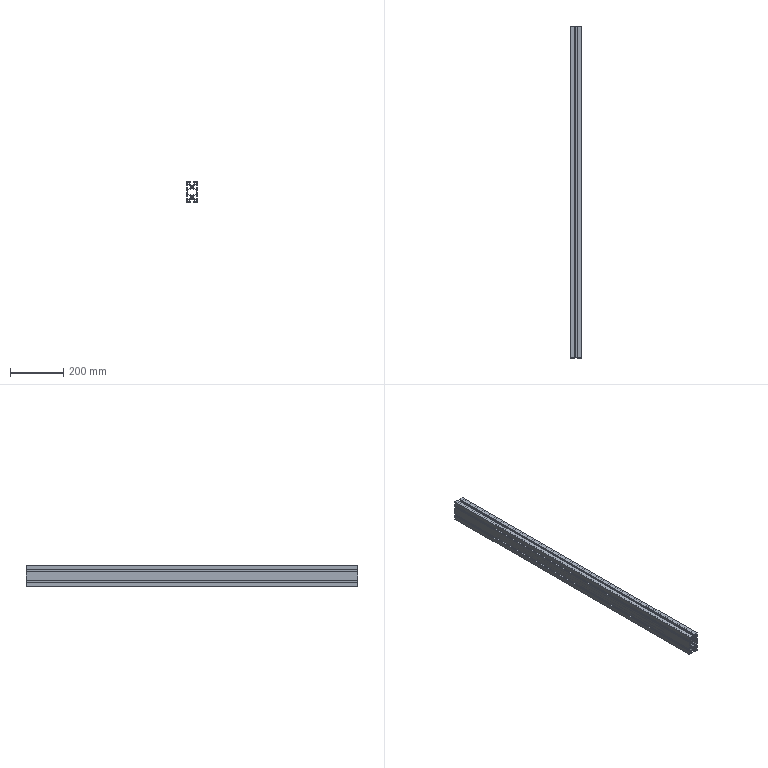Component | SolidWorks | 30-01A-1_EF4080-500-1 | 1 solid | 84 faces | box 40 x 1250 x 80 mm | volume 1438807 mm3 | plane 58 | cylinder 26 | commonest cylinder face diameters 8 x12 19 x10 6.8 x4
build123d program:
from build123d import *

# Parameters (mm, degrees)
SKETCH1_R      = 4
SKETCH1_R_2    = 3.4
EXTRUDE1_DEPTH = 625


with BuildPart() as part:
    # Sketch1 → Extrude1 (new, symmetric)
    with BuildSketch(Plane(origin=(0, 0, 0), x_dir=(0, 0, -1), z_dir=(0, 1, 0))):
        with BuildLine():
            Line((-40, 20), (-24.2, 20))
            Line((-24.2, 20), (-24.2, 16))
            Line((-24.2, 16), (-27.25, 16))
            Line((-27.25, 16), (-27.25, 9.361))
            ThreePointArc((-27.25, 9.361), (-20, 6), (-12.75, 9.361))
            Line((-12.75, 9.361), (-12.75, 16))
            Line((-12.75, 16), (-15.8, 16))
            Line((-15.8, 16), (-15.8, 20))
            Line((-15.8, 20), (15.8, 20))
            Line((15.8, 20), (15.8, 16))
            Line((15.8, 16), (12.75, 16))
            Line((12.75, 16), (12.75, 9.361))
            ThreePointArc((12.75, 9.361), (20, 6), (27.25, 9.361))
            Line((27.25, 9.361), (27.25, 16))
            Line((27.25, 16), (24.2, 16))
            Line((24.2, 16), (24.2, 20))
            Line((24.2, 20), (40, 20))
            Line((40, 20), (40, 4.2))
            Line((40, 4.2), (36, 4.2))
            Line((36, 4.2), (36, 7.25))
            Line((36, 7.25), (29.361, 7.25))
            ThreePointArc((29.361, 7.25), (26, 0), (29.361, -7.25))
            Line((29.361, -7.25), (36, -7.25))
            Line((36, -7.25), (36, -4.2))
            Line((36, -4.2), (40, -4.2))
            Line((40, -4.2), (40, -20))
            Line((40, -20), (24.2, -20))
            Line((24.2, -20), (24.2, -16))
            Line((24.2, -16), (27.25, -16))
            Line((27.25, -16), (27.25, -9.361))
            ThreePointArc((27.25, -9.361), (20, -6), (12.75, -9.361))
            Line((12.75, -9.361), (12.75, -16))
            Line((12.75, -16), (15.8, -16))
            Line((15.8, -16), (15.8, -20))
            Line((15.8, -20), (-15.8, -20))
            Line((-15.8, -20), (-15.8, -16))
            Line((-15.8, -16), (-12.75, -16))
            Line((-12.75, -16), (-12.75, -9.361))
            ThreePointArc((-12.75, -9.361), (-20, -6), (-27.25, -9.361))
            Line((-27.25, -9.361), (-27.25, -16))
            Line((-27.25, -16), (-24.2, -16))
            Line((-24.2, -16), (-24.2, -20))
            Line((-24.2, -20), (-40, -20))
            Line((-40, -20), (-40, -4.2))
            Line((-40, -4.2), (-36, -4.2))
            Line((-36, -4.2), (-36, -7.25))
            Line((-36, -7.25), (-29.361, -7.25))
            ThreePointArc((-29.361, -7.25), (-26, 0), (-29.361, 7.25))
            Line((-29.361, 7.25), (-36, 7.25))
            Line((-36, 7.25), (-36, 4.2))
            Line((-36, 4.2), (-40, 4.2))
            Line((-40, 4.2), (-40, 20))
        make_face()
        with Locations(Location((-33.5, 13.5, 0), (0, 0, 180))):
            Circle(SKETCH1_R, mode=Mode.SUBTRACT)
        with Locations(Location((-20, 0, 0), (0, 0, 180))):
            Circle(SKETCH1_R_2, mode=Mode.SUBTRACT)
        with Locations((-33.5, -13.5)):
            Circle(SKETCH1_R, mode=Mode.SUBTRACT)
        with Locations(Location((33.5, -13.5, 0), (0, 0, 180))):
            Circle(SKETCH1_R, mode=Mode.SUBTRACT)
        with Locations((20, 0)):
            Circle(SKETCH1_R_2, mode=Mode.SUBTRACT)
        with Locations((33.5, 13.5)):
            Circle(SKETCH1_R, mode=Mode.SUBTRACT)
        with BuildLine():
            Line((-10.5, -7.25), (-10.5, -13.5))
            ThreePointArc((-10.5, -13.5), (-9.328, -16.328), (-6.5, -17.5))
            Line((-6.5, -17.5), (6.5, -17.5))
            ThreePointArc((6.5, -17.5), (9.328, -16.328), (10.5, -13.5))
            Line((10.5, -13.5), (10.5, -7.25))
            Line((10.5, -7.25), (10.639, -7.25))
            ThreePointArc((10.639, -7.25), (14, 0), (10.639, 7.25))
            Line((10.639, 7.25), (10.5, 7.25))
            Line((10.5, 7.25), (10.5, 13.5))
            ThreePointArc((10.5, 13.5), (9.328, 16.328), (6.5, 17.5))
            Line((6.5, 17.5), (-6.5, 17.5))
            ThreePointArc((-6.5, 17.5), (-9.328, 16.328), (-10.5, 13.5))
            Line((-10.5, 13.5), (-10.5, 7.25))
            Line((-10.5, 7.25), (-10.639, 7.25))
            ThreePointArc((-10.639, 7.25), (-14, 0), (-10.639, -7.25))
            Line((-10.639, -7.25), (-10.5, -7.25))
        make_face(mode=Mode.SUBTRACT)
    extrude(amount=EXTRUDE1_DEPTH, both=True)


solid = part.part

# Placed as in the assembly
solid = solid.moved(Location((-427.43, 87.155, 0), (0, 0, 0)))